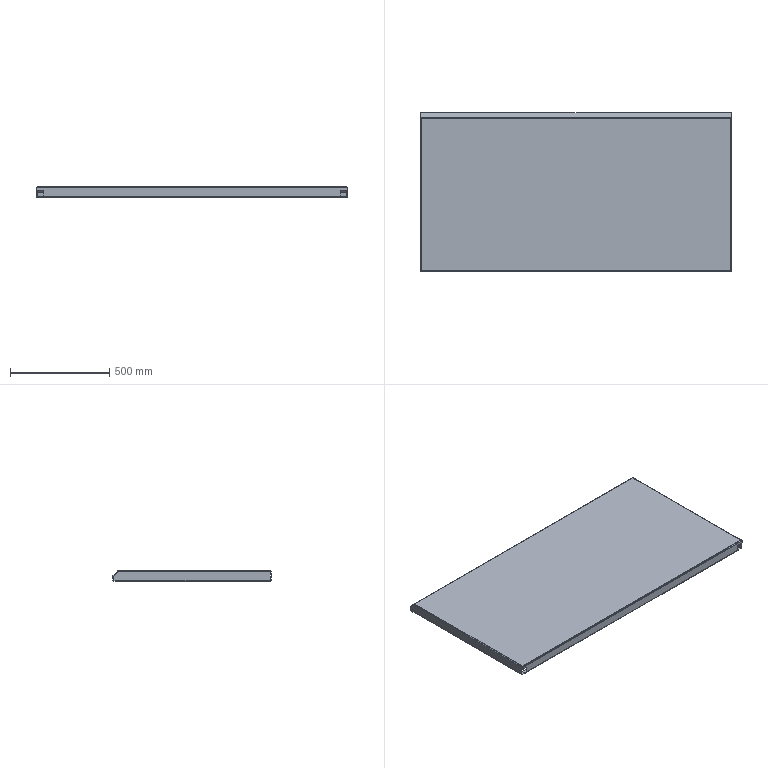Component | NX | DOOR | 1 solid | 84 faces | volume 3061202 mm3 | plane 64 | cylinder 20 | commonest cylinder face diameters 6 x11 10 x9